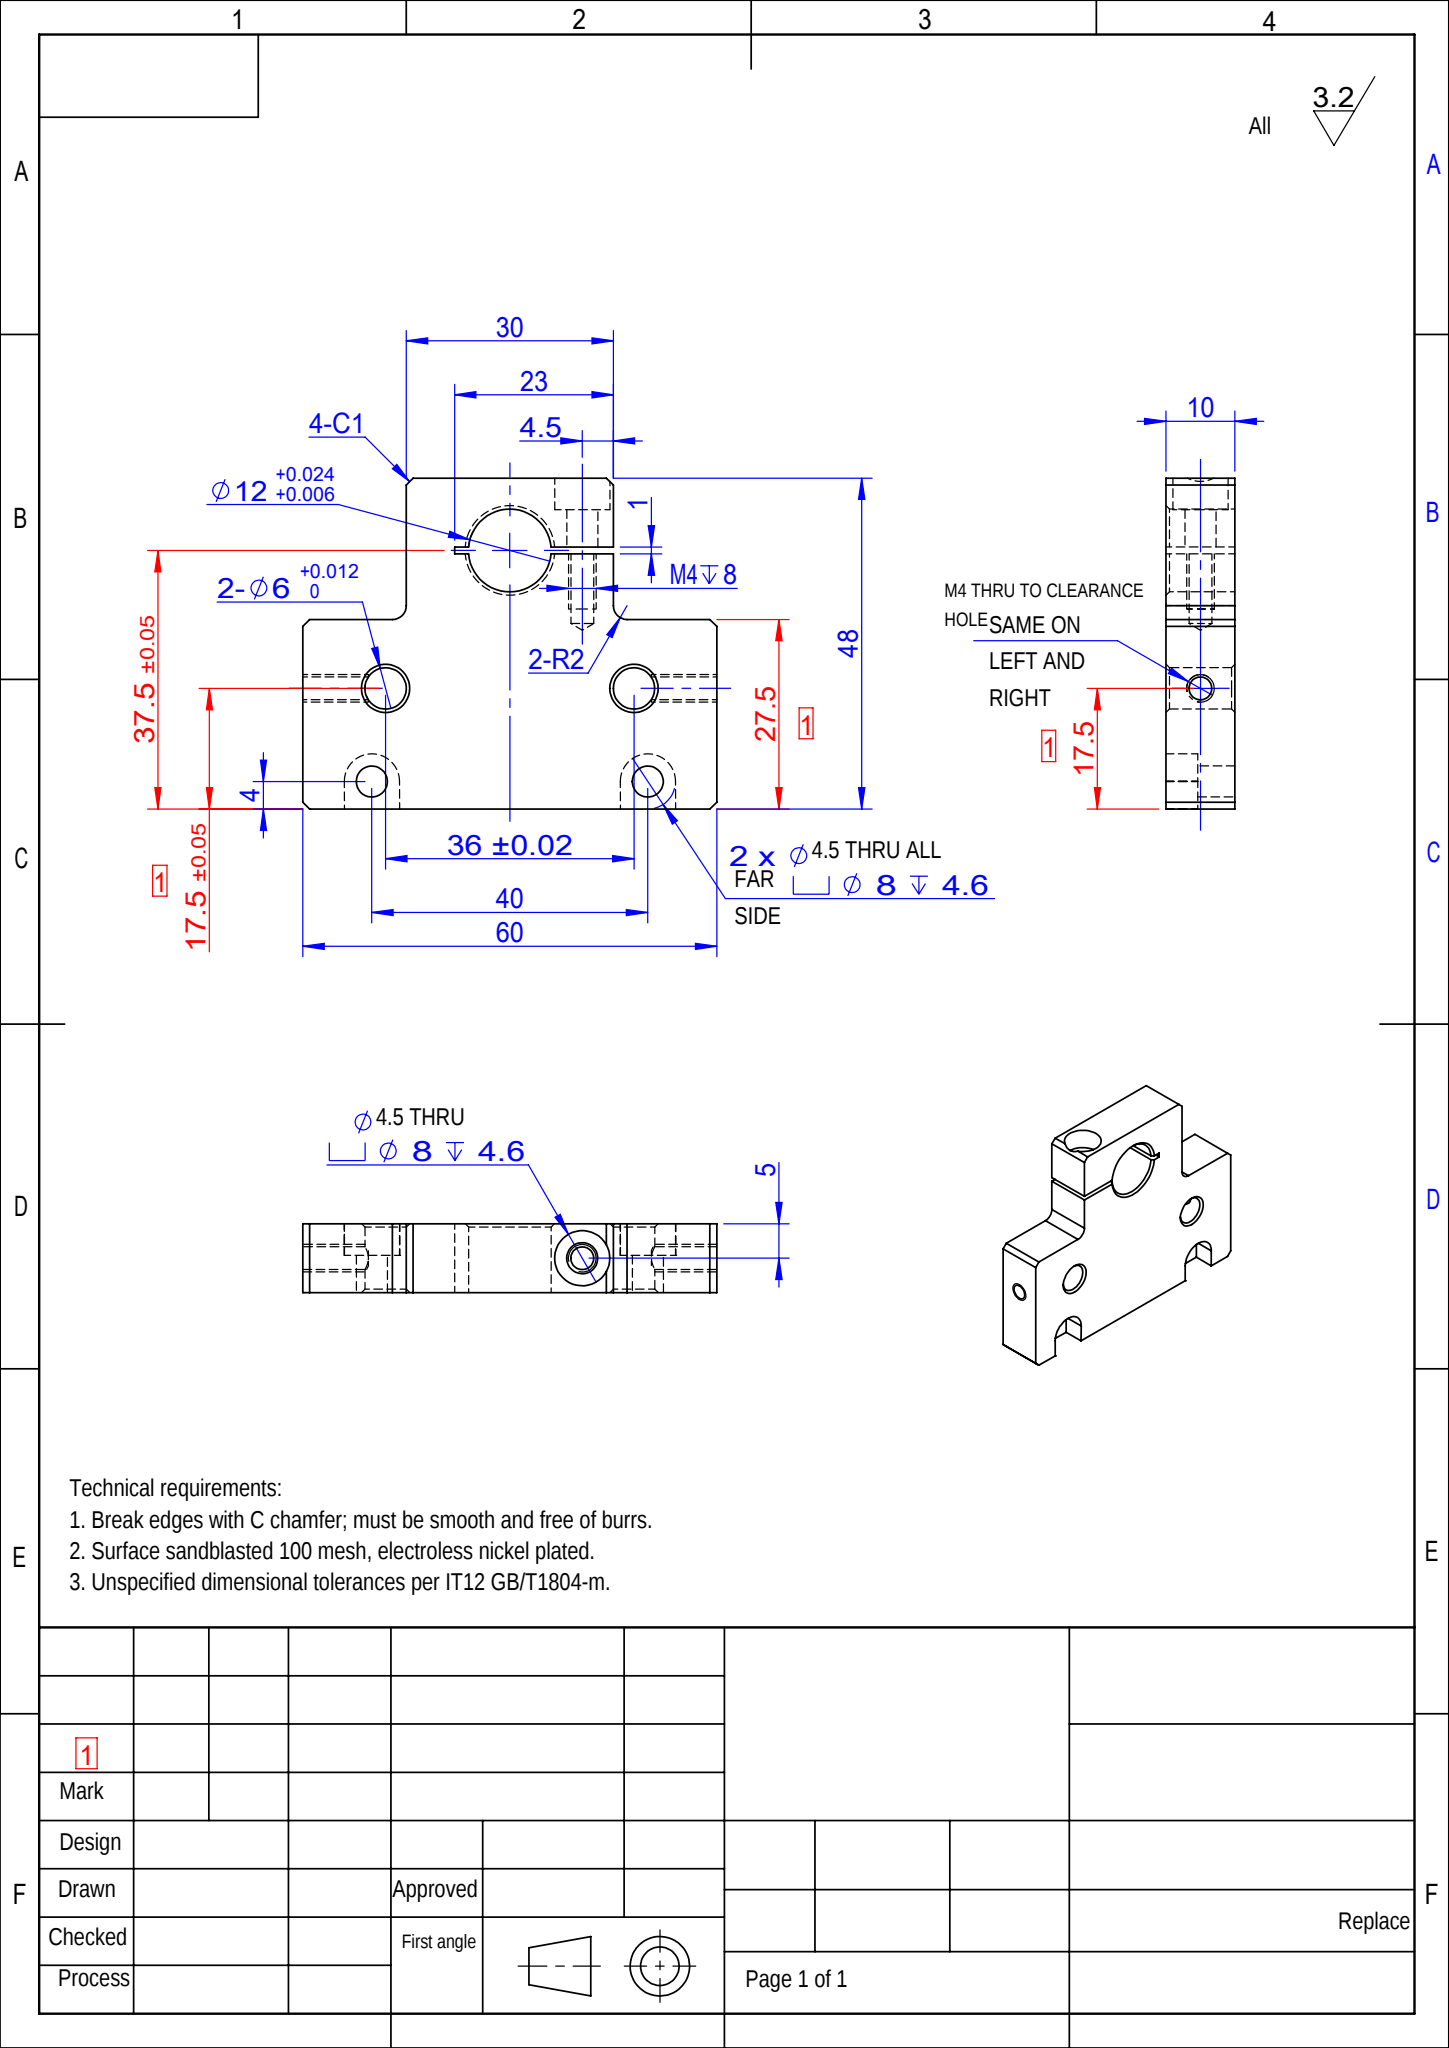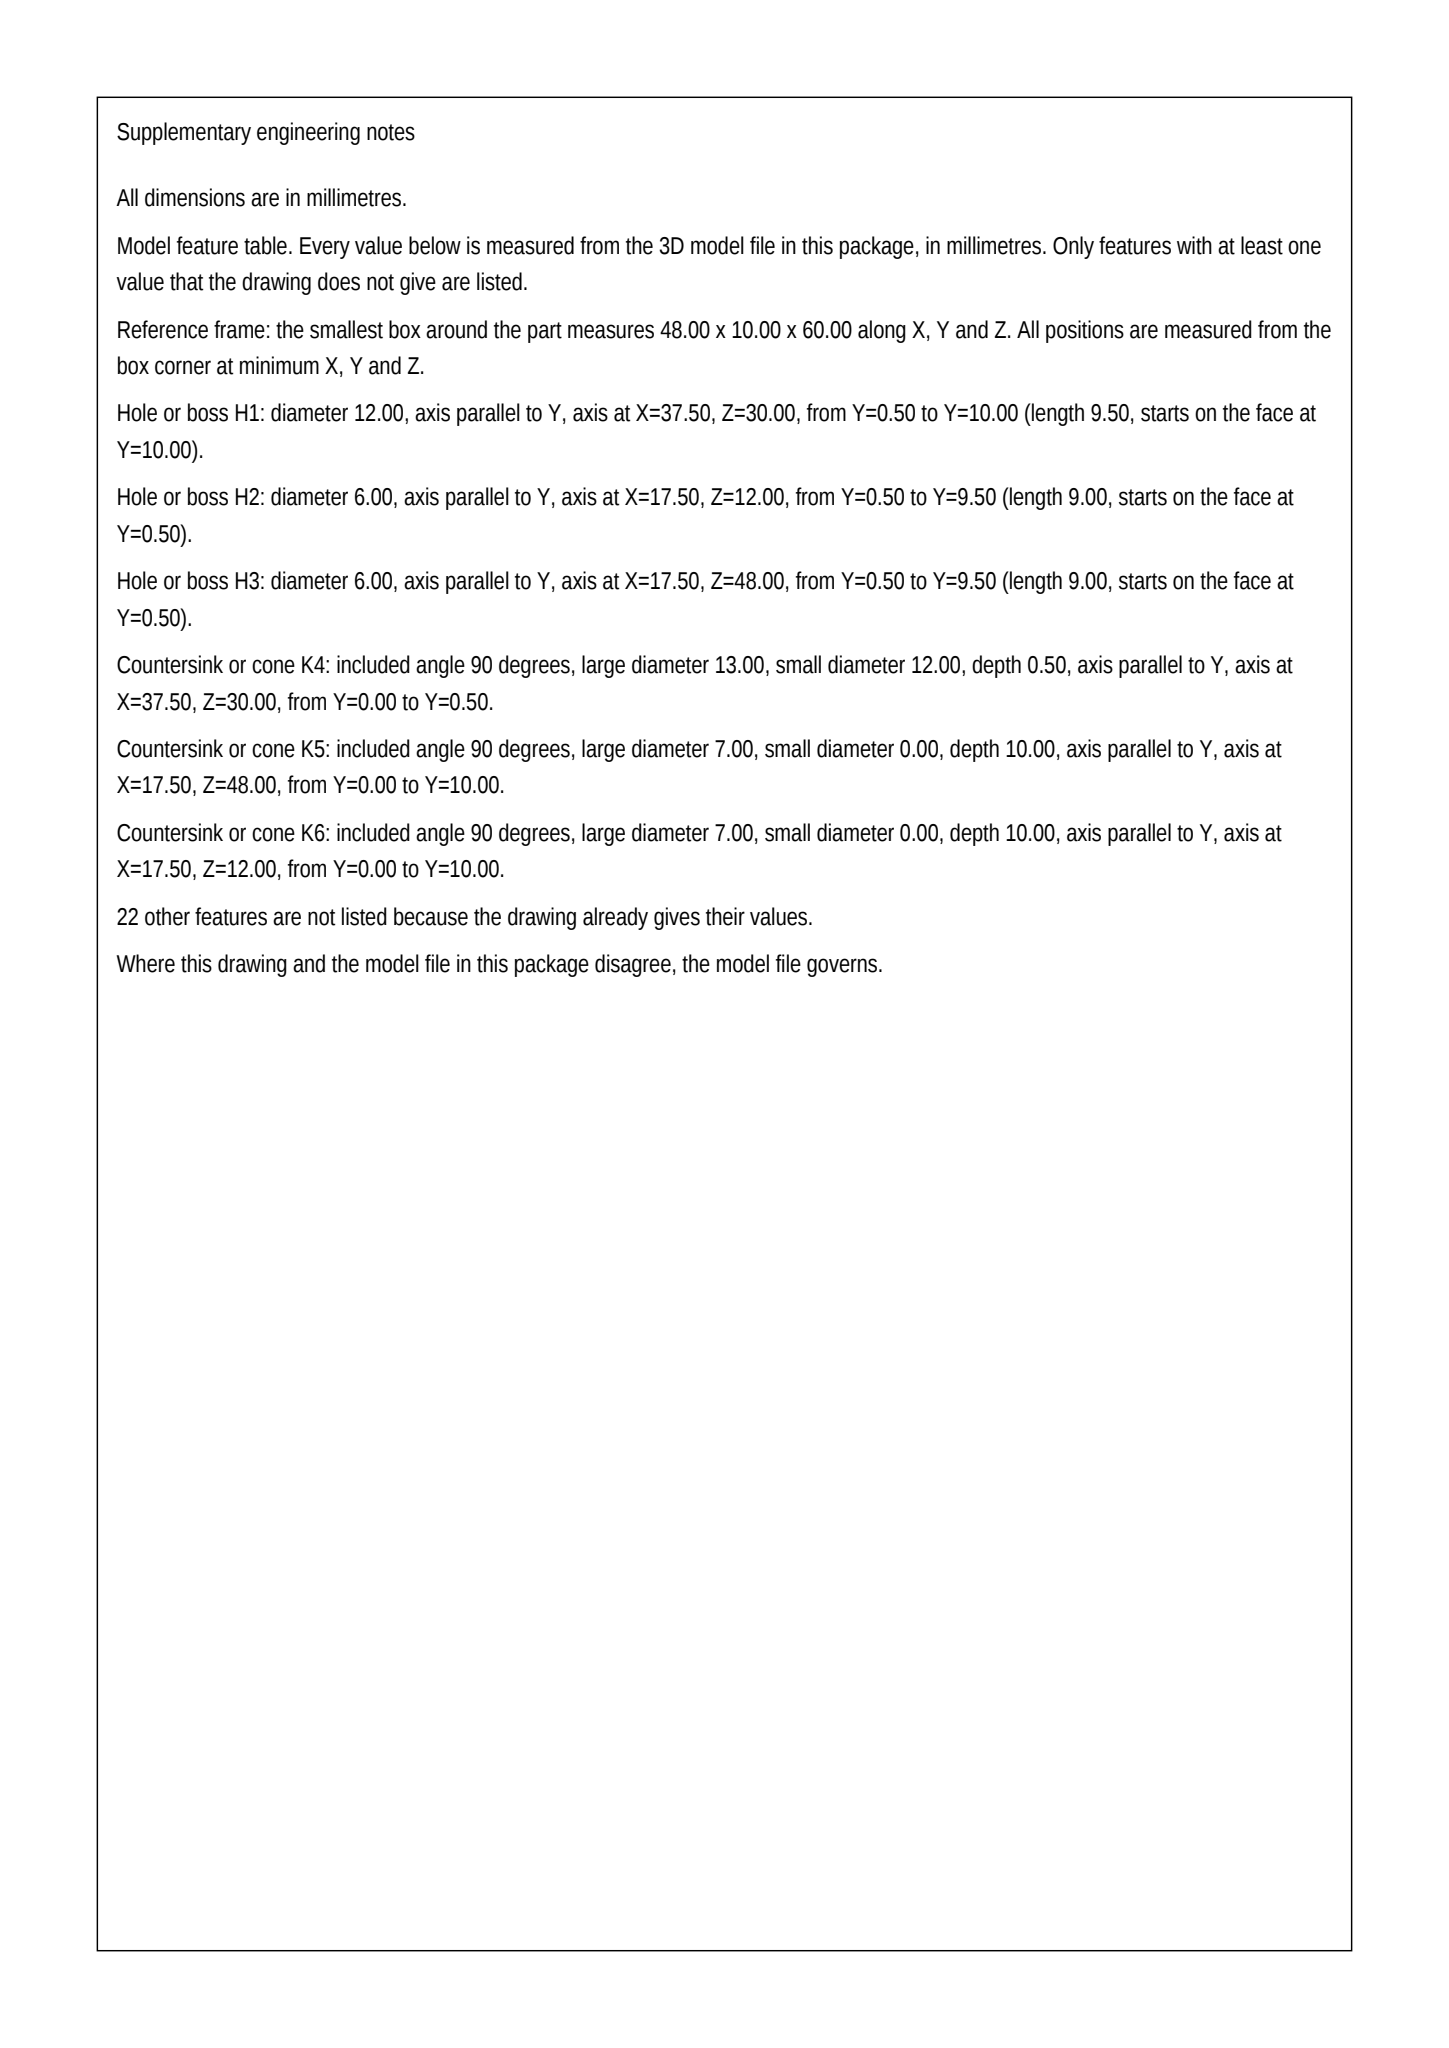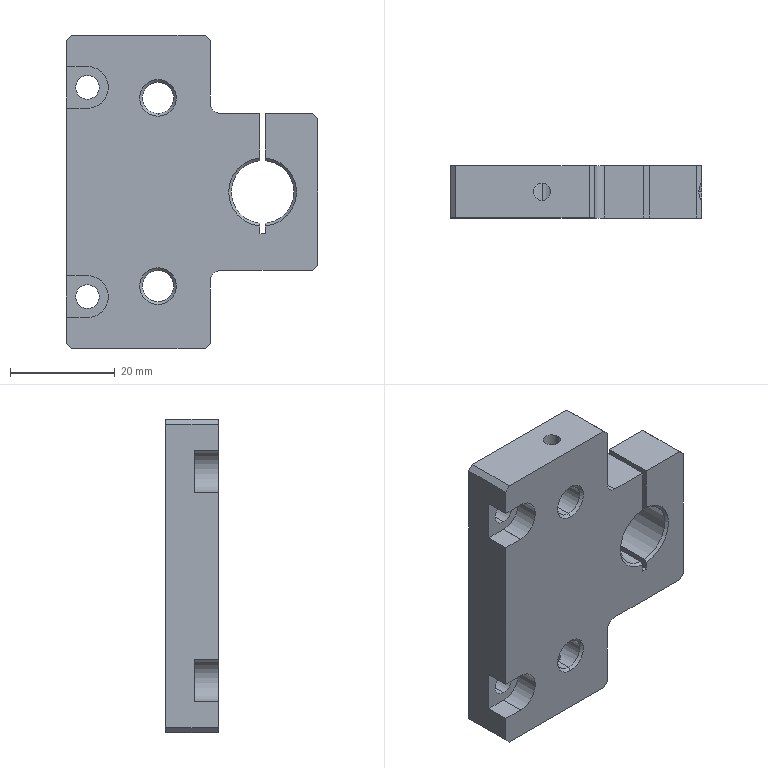Part | SolidWorks | mm | 1 solid | 69 faces | box 48 x 10 x 60 mm | volume 19557 mm3 | plane 29 | cylinder 28 | cone 12 | commonest cylinder face diameters 8 x8 4.5 x6 3.3 x6 6 x4 12 x2 4 x2